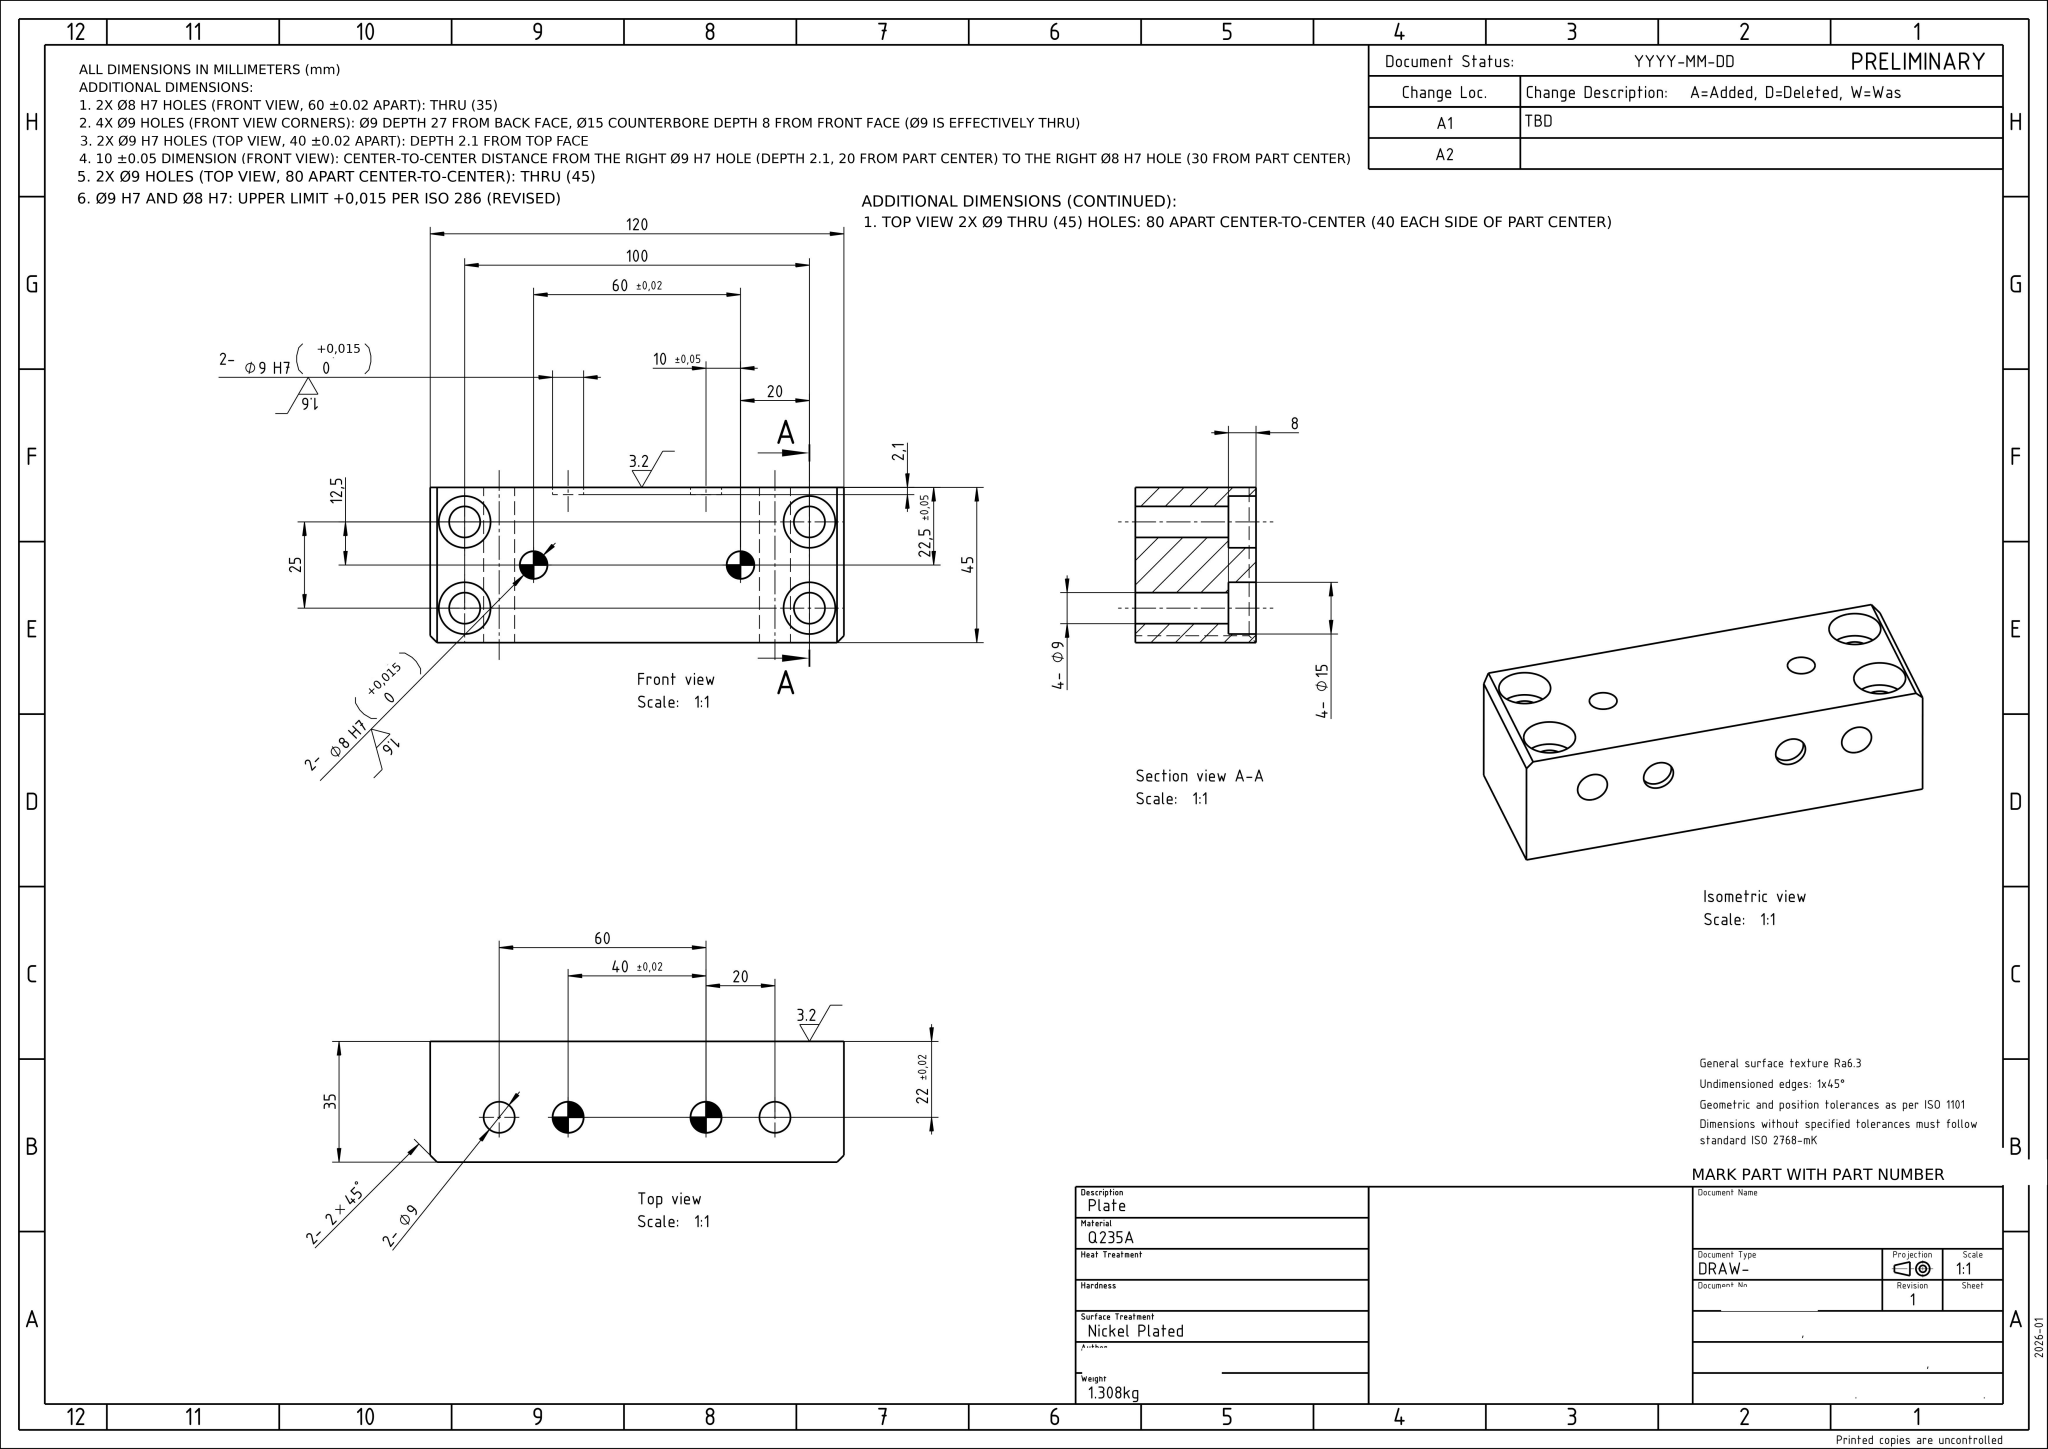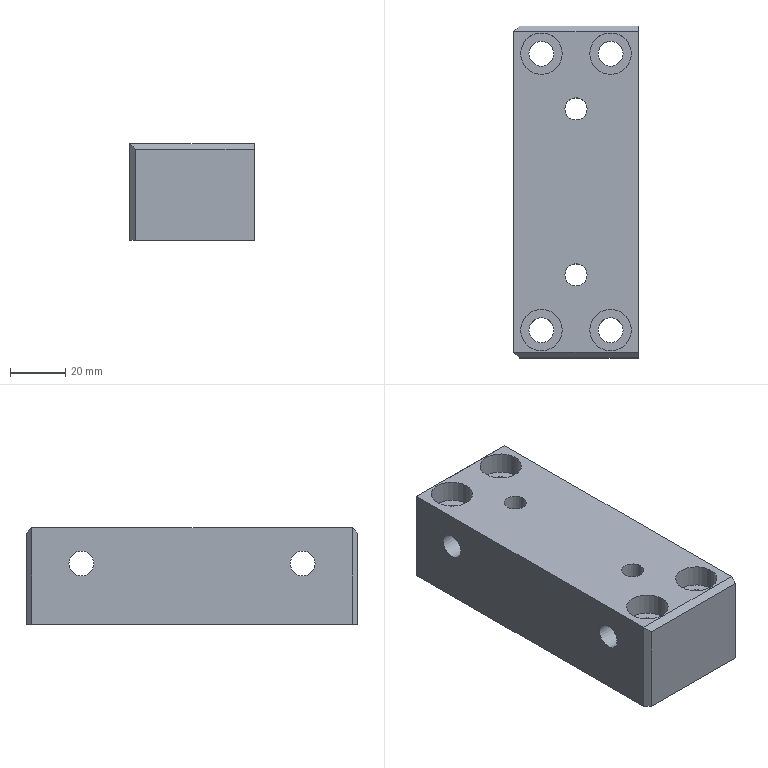Part | NX | mm | 1 solid | 30 faces | box 45 x 120 x 35 mm | volume 166648 mm3 | plane 16 | cylinder 14 | commonest cylinder face diameters 9 x8 15 x4 8 x2
STEP:
#1=CARTESIAN_POINT('',(0.,0.,0.));
#2=DIRECTION('',(0.,0.,1.));
#3=DIRECTION('',(1.,0.,0.));
#4=AXIS2_PLACEMENT_3D('',#1,#2,#3);
#5=(LENGTH_UNIT()NAMED_UNIT(*)SI_UNIT(.MILLI.,.METRE.));
#6=UNCERTAINTY_MEASURE_WITH_UNIT(LENGTH_MEASURE(0.00002),#5,'','');
#7=(NAMED_UNIT(*)PLANE_ANGLE_UNIT()SI_UNIT($,.RADIAN.));
#8=PLANE_ANGLE_MEASURE_WITH_UNIT(PLANE_ANGLE_MEASURE(0.01745),#7);
#9=DIMENSIONAL_EXPONENTS(0.,0.,0.,0.,0.,0.,0.);
#10=(CONVERSION_BASED_UNIT('',#8)NAMED_UNIT(#9)PLANE_ANGLE_UNIT());
#11=(NAMED_UNIT(*)SI_UNIT($,.STERADIAN.)SOLID_ANGLE_UNIT());
#12=(GEOMETRIC_REPRESENTATION_CONTEXT(3)GLOBAL_UNCERTAINTY_ASSIGNED_CONTEXT((#6))GLOBAL_UNIT_ASSIGNED_CONTEXT((#5,#10,#11))REPRESENTATION_CONTEXT('',''));
#13=SHAPE_REPRESENTATION('',(#4),#12);
#14=CARTESIAN_POINT('',(-22.5,44.5,22.));
#15=VERTEX_POINT('',#14);
#16=CARTESIAN_POINT('',(-22.5,40.,22.));
#17=DIRECTION('',(1.,-0.,0.));
#18=DIRECTION('',(0.,1.,0.));
#19=AXIS2_PLACEMENT_3D('',#16,#17,#18);
#20=CIRCLE('',#19,4.5);
#21=EDGE_CURVE('',#15,#15,#20,.T.);
#22=ORIENTED_EDGE('',*,*,#21,.T.);
#23=EDGE_LOOP('',(#22));
#24=FACE_BOUND('',#23,.T.);
#25=CARTESIAN_POINT('',(-22.5,-35.5,22.));
#26=VERTEX_POINT('',#25);
#27=CARTESIAN_POINT('',(-22.5,-40.,22.));
#28=DIRECTION('',(1.,-0.,0.));
#29=DIRECTION('',(0.,1.,0.));
#30=AXIS2_PLACEMENT_3D('',#27,#28,#29);
#31=CIRCLE('',#30,4.5);
#32=EDGE_CURVE('',#26,#26,#31,.T.);
#33=ORIENTED_EDGE('',*,*,#32,.T.);
#34=EDGE_LOOP('',(#33));
#35=FACE_BOUND('',#34,.T.);
#36=CARTESIAN_POINT('',(-22.5,58.,35.));
#37=VERTEX_POINT('',#36);
#38=CARTESIAN_POINT('',(-22.5,-58.,35.));
#39=VERTEX_POINT('',#38);
#40=CARTESIAN_POINT('',(-22.5,60.,35.));
#41=DIRECTION('',(-0.,-1.,0.));
#42=VECTOR('',#41,1.);
#43=LINE('',#40,#42);
#44=EDGE_CURVE('',#37,#39,#43,.T.);
#45=ORIENTED_EDGE('',*,*,#44,.F.);
#46=CARTESIAN_POINT('',(-22.5,58.,0.));
#47=VERTEX_POINT('',#46);
#48=CARTESIAN_POINT('',(-22.5,58.,35.));
#49=DIRECTION('',(0.,0.,-1.));
#50=VECTOR('',#49,1.);
#51=LINE('',#48,#50);
#52=EDGE_CURVE('',#37,#47,#51,.T.);
#53=ORIENTED_EDGE('',*,*,#52,.T.);
#54=CARTESIAN_POINT('',(-22.5,-58.,0.));
#55=VERTEX_POINT('',#54);
#56=CARTESIAN_POINT('',(-22.5,60.,0.));
#57=DIRECTION('',(-0.,-1.,0.));
#58=VECTOR('',#57,1.);
#59=LINE('',#56,#58);
#60=EDGE_CURVE('',#47,#55,#59,.T.);
#61=ORIENTED_EDGE('',*,*,#60,.T.);
#62=CARTESIAN_POINT('',(-22.5,-58.,35.));
#63=DIRECTION('',(0.,0.,1.));
#64=VECTOR('',#63,1.);
#65=LINE('',#62,#64);
#66=EDGE_CURVE('',#55,#39,#65,.T.);
#67=ORIENTED_EDGE('',*,*,#66,.T.);
#68=EDGE_LOOP('',(#45,#53,#61,#67));
#69=FACE_BOUND('',#68,.T.);
#70=CARTESIAN_POINT('',(-22.5,60.,35.));
#71=DIRECTION('',(1.,-0.,0.));
#72=DIRECTION('',(0.,1.,0.));
#73=AXIS2_PLACEMENT_3D('',#70,#71,#72);
#74=PLANE('',#73);
#75=ADVANCED_FACE('',(#24,#35,#69),#74,.F.);
#76=CARTESIAN_POINT('',(22.5,-60.,33.));
#77=VERTEX_POINT('',#76);
#78=CARTESIAN_POINT('',(22.5,-60.,0.));
#79=VERTEX_POINT('',#78);
#80=CARTESIAN_POINT('',(22.5,-60.,35.));
#81=DIRECTION('',(0.,0.,-1.));
#82=VECTOR('',#81,1.);
#83=LINE('',#80,#82);
#84=EDGE_CURVE('',#77,#79,#83,.T.);
#85=ORIENTED_EDGE('',*,*,#84,.F.);
#86=CARTESIAN_POINT('',(-20.5,-60.,33.));
#87=VERTEX_POINT('',#86);
#88=CARTESIAN_POINT('',(-22.5,-60.,33.));
#89=DIRECTION('',(-1.,-0.,0.));
#90=VECTOR('',#89,1.);
#91=LINE('',#88,#90);
#92=EDGE_CURVE('',#77,#87,#91,.T.);
#93=ORIENTED_EDGE('',*,*,#92,.T.);
#94=CARTESIAN_POINT('',(-20.5,-60.,0.));
#95=VERTEX_POINT('',#94);
#96=CARTESIAN_POINT('',(-20.5,-60.,35.));
#97=DIRECTION('',(0.,0.,-1.));
#98=VECTOR('',#97,1.);
#99=LINE('',#96,#98);
#100=EDGE_CURVE('',#87,#95,#99,.T.);
#101=ORIENTED_EDGE('',*,*,#100,.T.);
#102=CARTESIAN_POINT('',(-22.5,-60.,0.));
#103=DIRECTION('',(1.,0.,0.));
#104=VECTOR('',#103,1.);
#105=LINE('',#102,#104);
#106=EDGE_CURVE('',#95,#79,#105,.T.);
#107=ORIENTED_EDGE('',*,*,#106,.T.);
#108=EDGE_LOOP('',(#85,#93,#101,#107));
#109=FACE_OUTER_BOUND('',#108,.T.);
#110=CARTESIAN_POINT('',(-22.5,-60.,35.));
#111=DIRECTION('',(-0.,1.,0.));
#112=DIRECTION('',(-1.,-0.,0.));
#113=AXIS2_PLACEMENT_3D('',#110,#111,#112);
#114=PLANE('',#113);
#115=ADVANCED_FACE('',(#109),#114,.F.);
#116=CARTESIAN_POINT('',(22.5,35.5,22.));
#117=VERTEX_POINT('',#116);
#118=CARTESIAN_POINT('',(22.5,40.,22.));
#119=DIRECTION('',(-1.,0.,0.));
#120=DIRECTION('',(-0.,-1.,0.));
#121=AXIS2_PLACEMENT_3D('',#118,#119,#120);
#122=CIRCLE('',#121,4.5);
#123=EDGE_CURVE('',#117,#117,#122,.T.);
#124=ORIENTED_EDGE('',*,*,#123,.T.);
#125=EDGE_LOOP('',(#124));
#126=FACE_BOUND('',#125,.T.);
#127=CARTESIAN_POINT('',(22.5,-44.5,22.));
#128=VERTEX_POINT('',#127);
#129=CARTESIAN_POINT('',(22.5,-40.,22.));
#130=DIRECTION('',(-1.,0.,0.));
#131=DIRECTION('',(-0.,-1.,0.));
#132=AXIS2_PLACEMENT_3D('',#129,#130,#131);
#133=CIRCLE('',#132,4.5);
#134=EDGE_CURVE('',#128,#128,#133,.T.);
#135=ORIENTED_EDGE('',*,*,#134,.T.);
#136=EDGE_LOOP('',(#135));
#137=FACE_BOUND('',#136,.T.);
#138=CARTESIAN_POINT('',(22.5,15.5,22.));
#139=VERTEX_POINT('',#138);
#140=CARTESIAN_POINT('',(22.5,20.,22.));
#141=DIRECTION('',(-1.,0.,0.));
#142=DIRECTION('',(-0.,-1.,0.));
#143=AXIS2_PLACEMENT_3D('',#140,#141,#142);
#144=CIRCLE('',#143,4.5);
#145=EDGE_CURVE('',#139,#139,#144,.T.);
#146=ORIENTED_EDGE('',*,*,#145,.T.);
#147=EDGE_LOOP('',(#146));
#148=FACE_BOUND('',#147,.T.);
#149=CARTESIAN_POINT('',(22.5,-24.5,22.));
#150=VERTEX_POINT('',#149);
#151=CARTESIAN_POINT('',(22.5,-20.,22.));
#152=DIRECTION('',(-1.,0.,0.));
#153=DIRECTION('',(-0.,-1.,0.));
#154=AXIS2_PLACEMENT_3D('',#151,#152,#153);
#155=CIRCLE('',#154,4.5);
#156=EDGE_CURVE('',#150,#150,#155,.T.);
#157=ORIENTED_EDGE('',*,*,#156,.T.);
#158=EDGE_LOOP('',(#157));
#159=FACE_BOUND('',#158,.T.);
#160=CARTESIAN_POINT('',(22.5,60.,33.));
#161=VERTEX_POINT('',#160);
#162=CARTESIAN_POINT('',(22.5,60.,0.));
#163=VERTEX_POINT('',#162);
#164=CARTESIAN_POINT('',(22.5,60.,35.));
#165=DIRECTION('',(0.,0.,-1.));
#166=VECTOR('',#165,1.);
#167=LINE('',#164,#166);
#168=EDGE_CURVE('',#161,#163,#167,.T.);
#169=ORIENTED_EDGE('',*,*,#168,.F.);
#170=CARTESIAN_POINT('',(22.5,58.,35.));
#171=VERTEX_POINT('',#170);
#172=CARTESIAN_POINT('',(22.5,58.,35.));
#173=DIRECTION('',(-0.,-0.7071,0.7071));
#174=VECTOR('',#173,1.);
#175=LINE('',#172,#174);
#176=EDGE_CURVE('',#161,#171,#175,.T.);
#177=ORIENTED_EDGE('',*,*,#176,.T.);
#178=CARTESIAN_POINT('',(22.5,-58.,35.));
#179=VERTEX_POINT('',#178);
#180=CARTESIAN_POINT('',(22.5,-60.,35.));
#181=DIRECTION('',(0.,1.,0.));
#182=VECTOR('',#181,1.);
#183=LINE('',#180,#182);
#184=EDGE_CURVE('',#179,#171,#183,.T.);
#185=ORIENTED_EDGE('',*,*,#184,.F.);
#186=CARTESIAN_POINT('',(22.5,-58.,35.));
#187=DIRECTION('',(-0.,-0.7071,-0.7071));
#188=VECTOR('',#187,1.);
#189=LINE('',#186,#188);
#190=EDGE_CURVE('',#179,#77,#189,.T.);
#191=ORIENTED_EDGE('',*,*,#190,.T.);
#192=ORIENTED_EDGE('',*,*,#84,.T.);
#193=CARTESIAN_POINT('',(22.5,-60.,0.));
#194=DIRECTION('',(0.,1.,0.));
#195=VECTOR('',#194,1.);
#196=LINE('',#193,#195);
#197=EDGE_CURVE('',#79,#163,#196,.T.);
#198=ORIENTED_EDGE('',*,*,#197,.T.);
#199=EDGE_LOOP('',(#169,#177,#185,#191,#192,#198));
#200=FACE_BOUND('',#199,.T.);
#201=CARTESIAN_POINT('',(22.5,-60.,35.));
#202=DIRECTION('',(-1.,0.,0.));
#203=DIRECTION('',(-0.,-1.,0.));
#204=AXIS2_PLACEMENT_3D('',#201,#202,#203);
#205=PLANE('',#204);
#206=ADVANCED_FACE('',(#126,#137,#148,#159,#200),#205,.F.);
#207=CARTESIAN_POINT('',(-20.5,60.,0.));
#208=VERTEX_POINT('',#207);
#209=CARTESIAN_POINT('',(22.5,60.,0.));
#210=DIRECTION('',(-1.,-0.,0.));
#211=VECTOR('',#210,1.);
#212=LINE('',#209,#211);
#213=EDGE_CURVE('',#163,#208,#212,.T.);
#214=ORIENTED_EDGE('',*,*,#213,.T.);
#215=CARTESIAN_POINT('',(-20.5,60.,33.));
#216=VERTEX_POINT('',#215);
#217=CARTESIAN_POINT('',(-20.5,60.,35.));
#218=DIRECTION('',(0.,0.,1.));
#219=VECTOR('',#218,1.);
#220=LINE('',#217,#219);
#221=EDGE_CURVE('',#208,#216,#220,.T.);
#222=ORIENTED_EDGE('',*,*,#221,.T.);
#223=CARTESIAN_POINT('',(22.5,60.,33.));
#224=DIRECTION('',(1.,0.,0.));
#225=VECTOR('',#224,1.);
#226=LINE('',#223,#225);
#227=EDGE_CURVE('',#216,#161,#226,.T.);
#228=ORIENTED_EDGE('',*,*,#227,.T.);
#229=ORIENTED_EDGE('',*,*,#168,.T.);
#230=EDGE_LOOP('',(#214,#222,#228,#229));
#231=FACE_OUTER_BOUND('',#230,.T.);
#232=CARTESIAN_POINT('',(22.5,60.,35.));
#233=DIRECTION('',(0.,-1.,0.));
#234=DIRECTION('',(1.,0.,0.));
#235=AXIS2_PLACEMENT_3D('',#232,#233,#234);
#236=PLANE('',#235);
#237=ADVANCED_FACE('',(#231),#236,.F.);
#238=CARTESIAN_POINT('',(5.,50.,35.));
#239=VERTEX_POINT('',#238);
#240=CARTESIAN_POINT('',(12.5,50.,35.));
#241=DIRECTION('',(0.,0.,-1.));
#242=DIRECTION('',(-1.,0.,0.));
#243=AXIS2_PLACEMENT_3D('',#240,#241,#242);
#244=CIRCLE('',#243,7.5);
#245=EDGE_CURVE('',#239,#239,#244,.T.);
#246=ORIENTED_EDGE('',*,*,#245,.T.);
#247=EDGE_LOOP('',(#246));
#248=FACE_BOUND('',#247,.T.);
#249=CARTESIAN_POINT('',(5.,-50.,35.));
#250=VERTEX_POINT('',#249);
#251=CARTESIAN_POINT('',(12.5,-50.,35.));
#252=DIRECTION('',(0.,0.,-1.));
#253=DIRECTION('',(-1.,0.,0.));
#254=AXIS2_PLACEMENT_3D('',#251,#252,#253);
#255=CIRCLE('',#254,7.5);
#256=EDGE_CURVE('',#250,#250,#255,.T.);
#257=ORIENTED_EDGE('',*,*,#256,.T.);
#258=EDGE_LOOP('',(#257));
#259=FACE_BOUND('',#258,.T.);
#260=CARTESIAN_POINT('',(-20.,50.,35.));
#261=VERTEX_POINT('',#260);
#262=CARTESIAN_POINT('',(-12.5,50.,35.));
#263=DIRECTION('',(0.,0.,-1.));
#264=DIRECTION('',(-1.,0.,0.));
#265=AXIS2_PLACEMENT_3D('',#262,#263,#264);
#266=CIRCLE('',#265,7.5);
#267=EDGE_CURVE('',#261,#261,#266,.T.);
#268=ORIENTED_EDGE('',*,*,#267,.T.);
#269=EDGE_LOOP('',(#268));
#270=FACE_BOUND('',#269,.T.);
#271=CARTESIAN_POINT('',(-20.,-50.,35.));
#272=VERTEX_POINT('',#271);
#273=CARTESIAN_POINT('',(-12.5,-50.,35.));
#274=DIRECTION('',(0.,0.,-1.));
#275=DIRECTION('',(-1.,0.,0.));
#276=AXIS2_PLACEMENT_3D('',#273,#274,#275);
#277=CIRCLE('',#276,7.5);
#278=EDGE_CURVE('',#272,#272,#277,.T.);
#279=ORIENTED_EDGE('',*,*,#278,.T.);
#280=EDGE_LOOP('',(#279));
#281=FACE_BOUND('',#280,.T.);
#282=CARTESIAN_POINT('',(-4.,30.,35.));
#283=VERTEX_POINT('',#282);
#284=CARTESIAN_POINT('',(0.,30.,35.));
#285=DIRECTION('',(0.,0.,-1.));
#286=DIRECTION('',(-1.,0.,0.));
#287=AXIS2_PLACEMENT_3D('',#284,#285,#286);
#288=CIRCLE('',#287,4.);
#289=EDGE_CURVE('',#283,#283,#288,.T.);
#290=ORIENTED_EDGE('',*,*,#289,.T.);
#291=EDGE_LOOP('',(#290));
#292=FACE_BOUND('',#291,.T.);
#293=CARTESIAN_POINT('',(-4.,-30.,35.));
#294=VERTEX_POINT('',#293);
#295=CARTESIAN_POINT('',(-0.,-30.,35.));
#296=DIRECTION('',(0.,0.,-1.));
#297=DIRECTION('',(-1.,0.,0.));
#298=AXIS2_PLACEMENT_3D('',#295,#296,#297);
#299=CIRCLE('',#298,4.);
#300=EDGE_CURVE('',#294,#294,#299,.T.);
#301=ORIENTED_EDGE('',*,*,#300,.T.);
#302=EDGE_LOOP('',(#301));
#303=FACE_BOUND('',#302,.T.);
#304=ORIENTED_EDGE('',*,*,#184,.T.);
#305=CARTESIAN_POINT('',(-22.5,58.,35.));
#306=DIRECTION('',(-1.,-0.,0.));
#307=VECTOR('',#306,1.);
#308=LINE('',#305,#307);
#309=EDGE_CURVE('',#171,#37,#308,.T.);
#310=ORIENTED_EDGE('',*,*,#309,.T.);
#311=ORIENTED_EDGE('',*,*,#44,.T.);
#312=CARTESIAN_POINT('',(22.5,-58.,35.));
#313=DIRECTION('',(1.,0.,0.));
#314=VECTOR('',#313,1.);
#315=LINE('',#312,#314);
#316=EDGE_CURVE('',#39,#179,#315,.T.);
#317=ORIENTED_EDGE('',*,*,#316,.T.);
#318=EDGE_LOOP('',(#304,#310,#311,#317));
#319=FACE_BOUND('',#318,.T.);
#320=CARTESIAN_POINT('',(0.,0.,35.));
#321=DIRECTION('',(0.,0.,1.));
#322=DIRECTION('',(1.,0.,0.));
#323=AXIS2_PLACEMENT_3D('',#320,#321,#322);
#324=PLANE('',#323);
#325=ADVANCED_FACE('',(#248,#259,#270,#281,#292,#303,#319),#324,.T.);
#326=CARTESIAN_POINT('',(17.,50.,0.));
#327=VERTEX_POINT('',#326);
#328=CARTESIAN_POINT('',(12.5,50.,0.));
#329=DIRECTION('',(0.,0.,1.));
#330=DIRECTION('',(1.,0.,0.));
#331=AXIS2_PLACEMENT_3D('',#328,#329,#330);
#332=CIRCLE('',#331,4.5);
#333=EDGE_CURVE('',#327,#327,#332,.T.);
#334=ORIENTED_EDGE('',*,*,#333,.T.);
#335=EDGE_LOOP('',(#334));
#336=FACE_BOUND('',#335,.T.);
#337=CARTESIAN_POINT('',(17.,-50.,0.));
#338=VERTEX_POINT('',#337);
#339=CARTESIAN_POINT('',(12.5,-50.,0.));
#340=DIRECTION('',(0.,0.,1.));
#341=DIRECTION('',(1.,0.,0.));
#342=AXIS2_PLACEMENT_3D('',#339,#340,#341);
#343=CIRCLE('',#342,4.5);
#344=EDGE_CURVE('',#338,#338,#343,.T.);
#345=ORIENTED_EDGE('',*,*,#344,.T.);
#346=EDGE_LOOP('',(#345));
#347=FACE_BOUND('',#346,.T.);
#348=CARTESIAN_POINT('',(-8.,50.,0.));
#349=VERTEX_POINT('',#348);
#350=CARTESIAN_POINT('',(-12.5,50.,0.));
#351=DIRECTION('',(0.,0.,1.));
#352=DIRECTION('',(1.,0.,0.));
#353=AXIS2_PLACEMENT_3D('',#350,#351,#352);
#354=CIRCLE('',#353,4.5);
#355=EDGE_CURVE('',#349,#349,#354,.T.);
#356=ORIENTED_EDGE('',*,*,#355,.T.);
#357=EDGE_LOOP('',(#356));
#358=FACE_BOUND('',#357,.T.);
#359=CARTESIAN_POINT('',(-8.,-50.,0.));
#360=VERTEX_POINT('',#359);
#361=CARTESIAN_POINT('',(-12.5,-50.,0.));
#362=DIRECTION('',(0.,0.,1.));
#363=DIRECTION('',(1.,0.,0.));
#364=AXIS2_PLACEMENT_3D('',#361,#362,#363);
#365=CIRCLE('',#364,4.5);
#366=EDGE_CURVE('',#360,#360,#365,.T.);
#367=ORIENTED_EDGE('',*,*,#366,.T.);
#368=EDGE_LOOP('',(#367));
#369=FACE_BOUND('',#368,.T.);
#370=CARTESIAN_POINT('',(4.,30.,0.));
#371=VERTEX_POINT('',#370);
#372=CARTESIAN_POINT('',(0.,30.,0.));
#373=DIRECTION('',(0.,0.,1.));
#374=DIRECTION('',(1.,0.,0.));
#375=AXIS2_PLACEMENT_3D('',#372,#373,#374);
#376=CIRCLE('',#375,4.);
#377=EDGE_CURVE('',#371,#371,#376,.T.);
#378=ORIENTED_EDGE('',*,*,#377,.T.);
#379=EDGE_LOOP('',(#378));
#380=FACE_BOUND('',#379,.T.);
#381=CARTESIAN_POINT('',(4.,-30.,0.));
#382=VERTEX_POINT('',#381);
#383=CARTESIAN_POINT('',(-0.,-30.,0.));
#384=DIRECTION('',(0.,0.,1.));
#385=DIRECTION('',(1.,0.,0.));
#386=AXIS2_PLACEMENT_3D('',#383,#384,#385);
#387=CIRCLE('',#386,4.);
#388=EDGE_CURVE('',#382,#382,#387,.T.);
#389=ORIENTED_EDGE('',*,*,#388,.T.);
#390=EDGE_LOOP('',(#389));
#391=FACE_BOUND('',#390,.T.);
#392=ORIENTED_EDGE('',*,*,#60,.F.);
#393=CARTESIAN_POINT('',(-22.5,58.,0.));
#394=DIRECTION('',(0.7071,0.7071,0.));
#395=VECTOR('',#394,1.);
#396=LINE('',#393,#395);
#397=EDGE_CURVE('',#47,#208,#396,.T.);
#398=ORIENTED_EDGE('',*,*,#397,.T.);
#399=ORIENTED_EDGE('',*,*,#213,.F.);
#400=ORIENTED_EDGE('',*,*,#197,.F.);
#401=ORIENTED_EDGE('',*,*,#106,.F.);
#402=CARTESIAN_POINT('',(-20.5,-60.,0.));
#403=DIRECTION('',(-0.7071,0.7071,0.));
#404=VECTOR('',#403,1.);
#405=LINE('',#402,#404);
#406=EDGE_CURVE('',#95,#55,#405,.T.);
#407=ORIENTED_EDGE('',*,*,#406,.T.);
#408=EDGE_LOOP('',(#392,#398,#399,#400,#401,#407));
#409=FACE_BOUND('',#408,.T.);
#410=CARTESIAN_POINT('',(0.,0.,0.));
#411=DIRECTION('',(0.,0.,1.));
#412=DIRECTION('',(1.,0.,0.));
#413=AXIS2_PLACEMENT_3D('',#410,#411,#412);
#414=PLANE('',#413);
#415=ADVANCED_FACE('',(#336,#347,#358,#369,#380,#391,#409),#414,.F.);
#416=ORIENTED_EDGE('',*,*,#176,.F.);
#417=ORIENTED_EDGE('',*,*,#227,.F.);
#418=CARTESIAN_POINT('',(-15.,65.5,27.5));
#419=DIRECTION('',(0.5774,0.5774,-0.5774));
#420=VECTOR('',#419,1.);
#421=LINE('',#418,#420);
#422=EDGE_CURVE('',#37,#216,#421,.T.);
#423=ORIENTED_EDGE('',*,*,#422,.F.);
#424=ORIENTED_EDGE('',*,*,#309,.F.);
#425=EDGE_LOOP('',(#416,#417,#423,#424));
#426=FACE_OUTER_BOUND('',#425,.T.);
#427=CARTESIAN_POINT('',(-0.,58.,35.));
#428=DIRECTION('',(-0.,0.7071,0.7071));
#429=DIRECTION('',(1.,0.,0.));
#430=AXIS2_PLACEMENT_3D('',#427,#428,#429);
#431=PLANE('',#430);
#432=ADVANCED_FACE('',(#426),#431,.T.);
#433=ORIENTED_EDGE('',*,*,#422,.T.);
#434=ORIENTED_EDGE('',*,*,#221,.F.);
#435=ORIENTED_EDGE('',*,*,#397,.F.);
#436=ORIENTED_EDGE('',*,*,#52,.F.);
#437=EDGE_LOOP('',(#433,#434,#435,#436));
#438=FACE_OUTER_BOUND('',#437,.T.);
#439=CARTESIAN_POINT('',(-22.5,58.,35.));
#440=DIRECTION('',(0.7071,-0.7071,0.));
#441=DIRECTION('',(0.,0.,-1.));
#442=AXIS2_PLACEMENT_3D('',#439,#440,#441);
#443=PLANE('',#442);
#444=ADVANCED_FACE('',(#438),#443,.F.);
#445=ORIENTED_EDGE('',*,*,#406,.F.);
#446=ORIENTED_EDGE('',*,*,#100,.F.);
#447=CARTESIAN_POINT('',(-21.167,-59.333,33.667));
#448=DIRECTION('',(0.5774,-0.5774,-0.5774));
#449=VECTOR('',#448,1.);
#450=LINE('',#447,#449);
#451=EDGE_CURVE('',#39,#87,#450,.T.);
#452=ORIENTED_EDGE('',*,*,#451,.F.);
#453=ORIENTED_EDGE('',*,*,#66,.F.);
#454=EDGE_LOOP('',(#445,#446,#452,#453));
#455=FACE_OUTER_BOUND('',#454,.T.);
#456=CARTESIAN_POINT('',(-20.5,-60.,35.));
#457=DIRECTION('',(0.7071,0.7071,0.));
#458=DIRECTION('',(0.,0.,-1.));
#459=AXIS2_PLACEMENT_3D('',#456,#457,#458);
#460=PLANE('',#459);
#461=ADVANCED_FACE('',(#455),#460,.F.);
#462=ORIENTED_EDGE('',*,*,#451,.T.);
#463=ORIENTED_EDGE('',*,*,#92,.F.);
#464=ORIENTED_EDGE('',*,*,#190,.F.);
#465=ORIENTED_EDGE('',*,*,#316,.F.);
#466=EDGE_LOOP('',(#462,#463,#464,#465));
#467=FACE_OUTER_BOUND('',#466,.T.);
#468=CARTESIAN_POINT('',(0.,-58.,35.));
#469=DIRECTION('',(0.,-0.7071,0.7071));
#470=DIRECTION('',(-1.,-0.,0.));
#471=AXIS2_PLACEMENT_3D('',#468,#469,#470);
#472=PLANE('',#471);
#473=ADVANCED_FACE('',(#467),#472,.T.);
#474=ORIENTED_EDGE('',*,*,#300,.F.);
#475=EDGE_LOOP('',(#474));
#476=FACE_BOUND('',#475,.T.);
#477=ORIENTED_EDGE('',*,*,#388,.F.);
#478=EDGE_LOOP('',(#477));
#479=FACE_BOUND('',#478,.T.);
#480=CARTESIAN_POINT('',(-0.,-30.,35.));
#481=DIRECTION('',(0.,0.,-1.));
#482=DIRECTION('',(-1.,0.,0.));
#483=AXIS2_PLACEMENT_3D('',#480,#481,#482);
#484=CYLINDRICAL_SURFACE('',#483,4.);
#485=ADVANCED_FACE('',(#476,#479),#484,.F.);
#486=ORIENTED_EDGE('',*,*,#289,.F.);
#487=EDGE_LOOP('',(#486));
#488=FACE_BOUND('',#487,.T.);
#489=ORIENTED_EDGE('',*,*,#377,.F.);
#490=EDGE_LOOP('',(#489));
#491=FACE_BOUND('',#490,.T.);
#492=CARTESIAN_POINT('',(0.,30.,35.));
#493=DIRECTION('',(0.,0.,-1.));
#494=DIRECTION('',(-1.,0.,0.));
#495=AXIS2_PLACEMENT_3D('',#492,#493,#494);
#496=CYLINDRICAL_SURFACE('',#495,4.);
#497=ADVANCED_FACE('',(#488,#491),#496,.F.);
#498=CARTESIAN_POINT('',(-17.,-50.,27.));
#499=VERTEX_POINT('',#498);
#500=CARTESIAN_POINT('',(-12.5,-50.,27.));
#501=DIRECTION('',(0.,0.,1.));
#502=DIRECTION('',(-1.,0.,0.));
#503=AXIS2_PLACEMENT_3D('',#500,#501,#502);
#504=CIRCLE('',#503,4.5);
#505=EDGE_CURVE('',#499,#499,#504,.T.);
#506=ORIENTED_EDGE('',*,*,#505,.T.);
#507=EDGE_LOOP('',(#506));
#508=FACE_BOUND('',#507,.T.);
#509=ORIENTED_EDGE('',*,*,#366,.F.);
#510=EDGE_LOOP('',(#509));
#511=FACE_BOUND('',#510,.T.);
#512=CARTESIAN_POINT('',(-12.5,-50.,-34.296));
#513=DIRECTION('',(0.,0.,-1.));
#514=DIRECTION('',(-1.,0.,0.));
#515=AXIS2_PLACEMENT_3D('',#512,#513,#514);
#516=CYLINDRICAL_SURFACE('',#515,4.5);
#517=ADVANCED_FACE('',(#508,#511),#516,.F.);
#518=ORIENTED_EDGE('',*,*,#505,.F.);
#519=EDGE_LOOP('',(#518));
#520=FACE_BOUND('',#519,.T.);
#521=CARTESIAN_POINT('',(-20.,-50.,27.));
#522=VERTEX_POINT('',#521);
#523=CARTESIAN_POINT('',(-12.5,-50.,27.));
#524=DIRECTION('',(0.,0.,1.));
#525=DIRECTION('',(-1.,0.,0.));
#526=AXIS2_PLACEMENT_3D('',#523,#524,#525);
#527=CIRCLE('',#526,7.5);
#528=EDGE_CURVE('',#522,#522,#527,.T.);
#529=ORIENTED_EDGE('',*,*,#528,.T.);
#530=EDGE_LOOP('',(#529));
#531=FACE_BOUND('',#530,.T.);
#532=CARTESIAN_POINT('',(-12.5,-50.,27.));
#533=DIRECTION('',(0.,0.,-1.));
#534=DIRECTION('',(-1.,0.,0.));
#535=AXIS2_PLACEMENT_3D('',#532,#533,#534);
#536=PLANE('',#535);
#537=ADVANCED_FACE('',(#520,#531),#536,.F.);
#538=ORIENTED_EDGE('',*,*,#528,.F.);
#539=EDGE_LOOP('',(#538));
#540=FACE_BOUND('',#539,.T.);
#541=ORIENTED_EDGE('',*,*,#278,.F.);
#542=EDGE_LOOP('',(#541));
#543=FACE_BOUND('',#542,.T.);
#544=CARTESIAN_POINT('',(-12.5,-50.,35.));
#545=DIRECTION('',(0.,0.,-1.));
#546=DIRECTION('',(-1.,0.,0.));
#547=AXIS2_PLACEMENT_3D('',#544,#545,#546);
#548=CYLINDRICAL_SURFACE('',#547,7.5);
#549=ADVANCED_FACE('',(#540,#543),#548,.F.);
#550=CARTESIAN_POINT('',(-17.,50.,27.));
#551=VERTEX_POINT('',#550);
#552=CARTESIAN_POINT('',(-12.5,50.,27.));
#553=DIRECTION('',(0.,0.,1.));
#554=DIRECTION('',(-1.,0.,0.));
#555=AXIS2_PLACEMENT_3D('',#552,#553,#554);
#556=CIRCLE('',#555,4.5);
#557=EDGE_CURVE('',#551,#551,#556,.T.);
#558=ORIENTED_EDGE('',*,*,#557,.T.);
#559=EDGE_LOOP('',(#558));
#560=FACE_BOUND('',#559,.T.);
#561=ORIENTED_EDGE('',*,*,#355,.F.);
#562=EDGE_LOOP('',(#561));
#563=FACE_BOUND('',#562,.T.);
#564=CARTESIAN_POINT('',(-12.5,50.,-34.296));
#565=DIRECTION('',(0.,0.,-1.));
#566=DIRECTION('',(-1.,0.,0.));
#567=AXIS2_PLACEMENT_3D('',#564,#565,#566);
#568=CYLINDRICAL_SURFACE('',#567,4.5);
#569=ADVANCED_FACE('',(#560,#563),#568,.F.);
#570=ORIENTED_EDGE('',*,*,#557,.F.);
#571=EDGE_LOOP('',(#570));
#572=FACE_BOUND('',#571,.T.);
#573=CARTESIAN_POINT('',(-20.,50.,27.));
#574=VERTEX_POINT('',#573);
#575=CARTESIAN_POINT('',(-12.5,50.,27.));
#576=DIRECTION('',(0.,0.,1.));
#577=DIRECTION('',(-1.,0.,0.));
#578=AXIS2_PLACEMENT_3D('',#575,#576,#577);
#579=CIRCLE('',#578,7.5);
#580=EDGE_CURVE('',#574,#574,#579,.T.);
#581=ORIENTED_EDGE('',*,*,#580,.T.);
#582=EDGE_LOOP('',(#581));
#583=FACE_BOUND('',#582,.T.);
#584=CARTESIAN_POINT('',(-12.5,50.,27.));
#585=DIRECTION('',(0.,0.,-1.));
#586=DIRECTION('',(-1.,0.,0.));
#587=AXIS2_PLACEMENT_3D('',#584,#585,#586);
#588=PLANE('',#587);
#589=ADVANCED_FACE('',(#572,#583),#588,.F.);
#590=ORIENTED_EDGE('',*,*,#580,.F.);
#591=EDGE_LOOP('',(#590));
#592=FACE_BOUND('',#591,.T.);
#593=ORIENTED_EDGE('',*,*,#267,.F.);
#594=EDGE_LOOP('',(#593));
#595=FACE_BOUND('',#594,.T.);
#596=CARTESIAN_POINT('',(-12.5,50.,35.));
#597=DIRECTION('',(0.,0.,-1.));
#598=DIRECTION('',(-1.,0.,0.));
#599=AXIS2_PLACEMENT_3D('',#596,#597,#598);
#600=CYLINDRICAL_SURFACE('',#599,7.5);
#601=ADVANCED_FACE('',(#592,#595),#600,.F.);
#602=CARTESIAN_POINT('',(8.,-50.,27.));
#603=VERTEX_POINT('',#602);
#604=CARTESIAN_POINT('',(12.5,-50.,27.));
#605=DIRECTION('',(0.,0.,1.));
#606=DIRECTION('',(-1.,0.,0.));
#607=AXIS2_PLACEMENT_3D('',#604,#605,#606);
#608=CIRCLE('',#607,4.5);
#609=EDGE_CURVE('',#603,#603,#608,.T.);
#610=ORIENTED_EDGE('',*,*,#609,.T.);
#611=EDGE_LOOP('',(#610));
#612=FACE_BOUND('',#611,.T.);
#613=ORIENTED_EDGE('',*,*,#344,.F.);
#614=EDGE_LOOP('',(#613));
#615=FACE_BOUND('',#614,.T.);
#616=CARTESIAN_POINT('',(12.5,-50.,-34.296));
#617=DIRECTION('',(0.,0.,-1.));
#618=DIRECTION('',(-1.,0.,0.));
#619=AXIS2_PLACEMENT_3D('',#616,#617,#618);
#620=CYLINDRICAL_SURFACE('',#619,4.5);
#621=ADVANCED_FACE('',(#612,#615),#620,.F.);
#622=ORIENTED_EDGE('',*,*,#609,.F.);
#623=EDGE_LOOP('',(#622));
#624=FACE_BOUND('',#623,.T.);
#625=CARTESIAN_POINT('',(5.,-50.,27.));
#626=VERTEX_POINT('',#625);
#627=CARTESIAN_POINT('',(12.5,-50.,27.));
#628=DIRECTION('',(0.,0.,1.));
#629=DIRECTION('',(-1.,0.,0.));
#630=AXIS2_PLACEMENT_3D('',#627,#628,#629);
#631=CIRCLE('',#630,7.5);
#632=EDGE_CURVE('',#626,#626,#631,.T.);
#633=ORIENTED_EDGE('',*,*,#632,.T.);
#634=EDGE_LOOP('',(#633));
#635=FACE_BOUND('',#634,.T.);
#636=CARTESIAN_POINT('',(12.5,-50.,27.));
#637=DIRECTION('',(0.,0.,-1.));
#638=DIRECTION('',(-1.,0.,0.));
#639=AXIS2_PLACEMENT_3D('',#636,#637,#638);
#640=PLANE('',#639);
#641=ADVANCED_FACE('',(#624,#635),#640,.F.);
#642=ORIENTED_EDGE('',*,*,#632,.F.);
#643=EDGE_LOOP('',(#642));
#644=FACE_BOUND('',#643,.T.);
#645=ORIENTED_EDGE('',*,*,#256,.F.);
#646=EDGE_LOOP('',(#645));
#647=FACE_BOUND('',#646,.T.);
#648=CARTESIAN_POINT('',(12.5,-50.,35.));
#649=DIRECTION('',(0.,0.,-1.));
#650=DIRECTION('',(-1.,0.,0.));
#651=AXIS2_PLACEMENT_3D('',#648,#649,#650);
#652=CYLINDRICAL_SURFACE('',#651,7.5);
#653=ADVANCED_FACE('',(#644,#647),#652,.F.);
#654=CARTESIAN_POINT('',(8.,50.,27.));
#655=VERTEX_POINT('',#654);
#656=CARTESIAN_POINT('',(12.5,50.,27.));
#657=DIRECTION('',(0.,0.,1.));
#658=DIRECTION('',(-1.,0.,0.));
#659=AXIS2_PLACEMENT_3D('',#656,#657,#658);
#660=CIRCLE('',#659,4.5);
#661=EDGE_CURVE('',#655,#655,#660,.T.);
#662=ORIENTED_EDGE('',*,*,#661,.T.);
#663=EDGE_LOOP('',(#662));
#664=FACE_BOUND('',#663,.T.);
#665=ORIENTED_EDGE('',*,*,#333,.F.);
#666=EDGE_LOOP('',(#665));
#667=FACE_BOUND('',#666,.T.);
#668=CARTESIAN_POINT('',(12.5,50.,-34.296));
#669=DIRECTION('',(0.,0.,-1.));
#670=DIRECTION('',(-1.,0.,0.));
#671=AXIS2_PLACEMENT_3D('',#668,#669,#670);
#672=CYLINDRICAL_SURFACE('',#671,4.5);
#673=ADVANCED_FACE('',(#664,#667),#672,.F.);
#674=ORIENTED_EDGE('',*,*,#661,.F.);
#675=EDGE_LOOP('',(#674));
#676=FACE_BOUND('',#675,.T.);
#677=CARTESIAN_POINT('',(5.,50.,27.));
#678=VERTEX_POINT('',#677);
#679=CARTESIAN_POINT('',(12.5,50.,27.));
#680=DIRECTION('',(0.,0.,1.));
#681=DIRECTION('',(-1.,0.,0.));
#682=AXIS2_PLACEMENT_3D('',#679,#680,#681);
#683=CIRCLE('',#682,7.5);
#684=EDGE_CURVE('',#678,#678,#683,.T.);
#685=ORIENTED_EDGE('',*,*,#684,.T.);
#686=EDGE_LOOP('',(#685));
#687=FACE_BOUND('',#686,.T.);
#688=CARTESIAN_POINT('',(12.5,50.,27.));
#689=DIRECTION('',(0.,0.,-1.));
#690=DIRECTION('',(-1.,0.,0.));
#691=AXIS2_PLACEMENT_3D('',#688,#689,#690);
#692=PLANE('',#691);
#693=ADVANCED_FACE('',(#676,#687),#692,.F.);
#694=ORIENTED_EDGE('',*,*,#684,.F.);
#695=EDGE_LOOP('',(#694));
#696=FACE_BOUND('',#695,.T.);
#697=ORIENTED_EDGE('',*,*,#245,.F.);
#698=EDGE_LOOP('',(#697));
#699=FACE_BOUND('',#698,.T.);
#700=CARTESIAN_POINT('',(12.5,50.,35.));
#701=DIRECTION('',(0.,0.,-1.));
#702=DIRECTION('',(-1.,0.,0.));
#703=AXIS2_PLACEMENT_3D('',#700,#701,#702);
#704=CYLINDRICAL_SURFACE('',#703,7.5);
#705=ADVANCED_FACE('',(#696,#699),#704,.F.);
#706=CARTESIAN_POINT('',(20.4,-24.5,22.));
#707=VERTEX_POINT('',#706);
#708=CARTESIAN_POINT('',(20.4,-20.,22.));
#709=DIRECTION('',(1.,-0.,0.));
#710=DIRECTION('',(-0.,-1.,0.));
#711=AXIS2_PLACEMENT_3D('',#708,#709,#710);
#712=CIRCLE('',#711,4.5);
#713=EDGE_CURVE('',#707,#707,#712,.T.);
#714=ORIENTED_EDGE('',*,*,#713,.T.);
#715=EDGE_LOOP('',(#714));
#716=FACE_OUTER_BOUND('',#715,.T.);
#717=CARTESIAN_POINT('',(20.4,-20.,22.));
#718=DIRECTION('',(-1.,0.,0.));
#719=DIRECTION('',(-0.,-1.,0.));
#720=AXIS2_PLACEMENT_3D('',#717,#718,#719);
#721=PLANE('',#720);
#722=ADVANCED_FACE('',(#716),#721,.F.);
#723=ORIENTED_EDGE('',*,*,#713,.F.);
#724=EDGE_LOOP('',(#723));
#725=FACE_BOUND('',#724,.T.);
#726=ORIENTED_EDGE('',*,*,#156,.F.);
#727=EDGE_LOOP('',(#726));
#728=FACE_BOUND('',#727,.T.);
#729=CARTESIAN_POINT('',(22.5,-20.,22.));
#730=DIRECTION('',(-1.,0.,0.));
#731=DIRECTION('',(-0.,-1.,0.));
#732=AXIS2_PLACEMENT_3D('',#729,#730,#731);
#733=CYLINDRICAL_SURFACE('',#732,4.5);
#734=ADVANCED_FACE('',(#725,#728),#733,.F.);
#735=CARTESIAN_POINT('',(20.4,15.5,22.));
#736=VERTEX_POINT('',#735);
#737=CARTESIAN_POINT('',(20.4,20.,22.));
#738=DIRECTION('',(1.,-0.,0.));
#739=DIRECTION('',(-0.,-1.,0.));
#740=AXIS2_PLACEMENT_3D('',#737,#738,#739);
#741=CIRCLE('',#740,4.5);
#742=EDGE_CURVE('',#736,#736,#741,.T.);
#743=ORIENTED_EDGE('',*,*,#742,.T.);
#744=EDGE_LOOP('',(#743));
#745=FACE_OUTER_BOUND('',#744,.T.);
#746=CARTESIAN_POINT('',(20.4,20.,22.));
#747=DIRECTION('',(-1.,0.,0.));
#748=DIRECTION('',(-0.,-1.,0.));
#749=AXIS2_PLACEMENT_3D('',#746,#747,#748);
#750=PLANE('',#749);
#751=ADVANCED_FACE('',(#745),#750,.F.);
#752=ORIENTED_EDGE('',*,*,#742,.F.);
#753=EDGE_LOOP('',(#752));
#754=FACE_BOUND('',#753,.T.);
#755=ORIENTED_EDGE('',*,*,#145,.F.);
#756=EDGE_LOOP('',(#755));
#757=FACE_BOUND('',#756,.T.);
#758=CARTESIAN_POINT('',(22.5,20.,22.));
#759=DIRECTION('',(-1.,0.,0.));
#760=DIRECTION('',(-0.,-1.,0.));
#761=AXIS2_PLACEMENT_3D('',#758,#759,#760);
#762=CYLINDRICAL_SURFACE('',#761,4.5);
#763=ADVANCED_FACE('',(#754,#757),#762,.F.);
#764=ORIENTED_EDGE('',*,*,#134,.F.);
#765=EDGE_LOOP('',(#764));
#766=FACE_BOUND('',#765,.T.);
#767=ORIENTED_EDGE('',*,*,#32,.F.);
#768=EDGE_LOOP('',(#767));
#769=FACE_BOUND('',#768,.T.);
#770=CARTESIAN_POINT('',(22.5,-40.,22.));
#771=DIRECTION('',(-1.,0.,0.));
#772=DIRECTION('',(-0.,-1.,0.));
#773=AXIS2_PLACEMENT_3D('',#770,#771,#772);
#774=CYLINDRICAL_SURFACE('',#773,4.5);
#775=ADVANCED_FACE('',(#766,#769),#774,.F.);
#776=ORIENTED_EDGE('',*,*,#123,.F.);
#777=EDGE_LOOP('',(#776));
#778=FACE_BOUND('',#777,.T.);
#779=ORIENTED_EDGE('',*,*,#21,.F.);
#780=EDGE_LOOP('',(#779));
#781=FACE_BOUND('',#780,.T.);
#782=CARTESIAN_POINT('',(22.5,40.,22.));
#783=DIRECTION('',(-1.,0.,0.));
#784=DIRECTION('',(-0.,-1.,0.));
#785=AXIS2_PLACEMENT_3D('',#782,#783,#784);
#786=CYLINDRICAL_SURFACE('',#785,4.5);
#787=ADVANCED_FACE('',(#778,#781),#786,.F.);
#788=CLOSED_SHELL('',(#75,#115,#206,#237,#325,#415,#432,#444,#461,#473,#485,#497,#517,#537,#549,#569,#589,#601,#621,#641,#653,#673,#693,#705,#722,#734,#751,#763,#775,#787));
#789=MANIFOLD_SOLID_BREP('',#788);
#790=ADVANCED_BREP_SHAPE_REPRESENTATION('',(#789),#12);
#791=SHAPE_REPRESENTATION_RELATIONSHIP('','',#13,#790);
#792=PRESENTATION_LAYER_ASSIGNMENT('','',(#789));
#793=COLOUR_RGB('',0.4,0.8,1.);
#794=FILL_AREA_STYLE_COLOUR('',#793);
#795=FILL_AREA_STYLE('',(#794));
#796=SURFACE_STYLE_FILL_AREA(#795);
#797=SURFACE_SIDE_STYLE('',(#796));
#798=SURFACE_STYLE_USAGE(.BOTH.,#797);
#799=PRESENTATION_STYLE_ASSIGNMENT((#798));
#800=STYLED_ITEM('',(#799),#789);
#801=MECHANICAL_DESIGN_GEOMETRIC_PRESENTATION_REPRESENTATION('',(#800),#12);